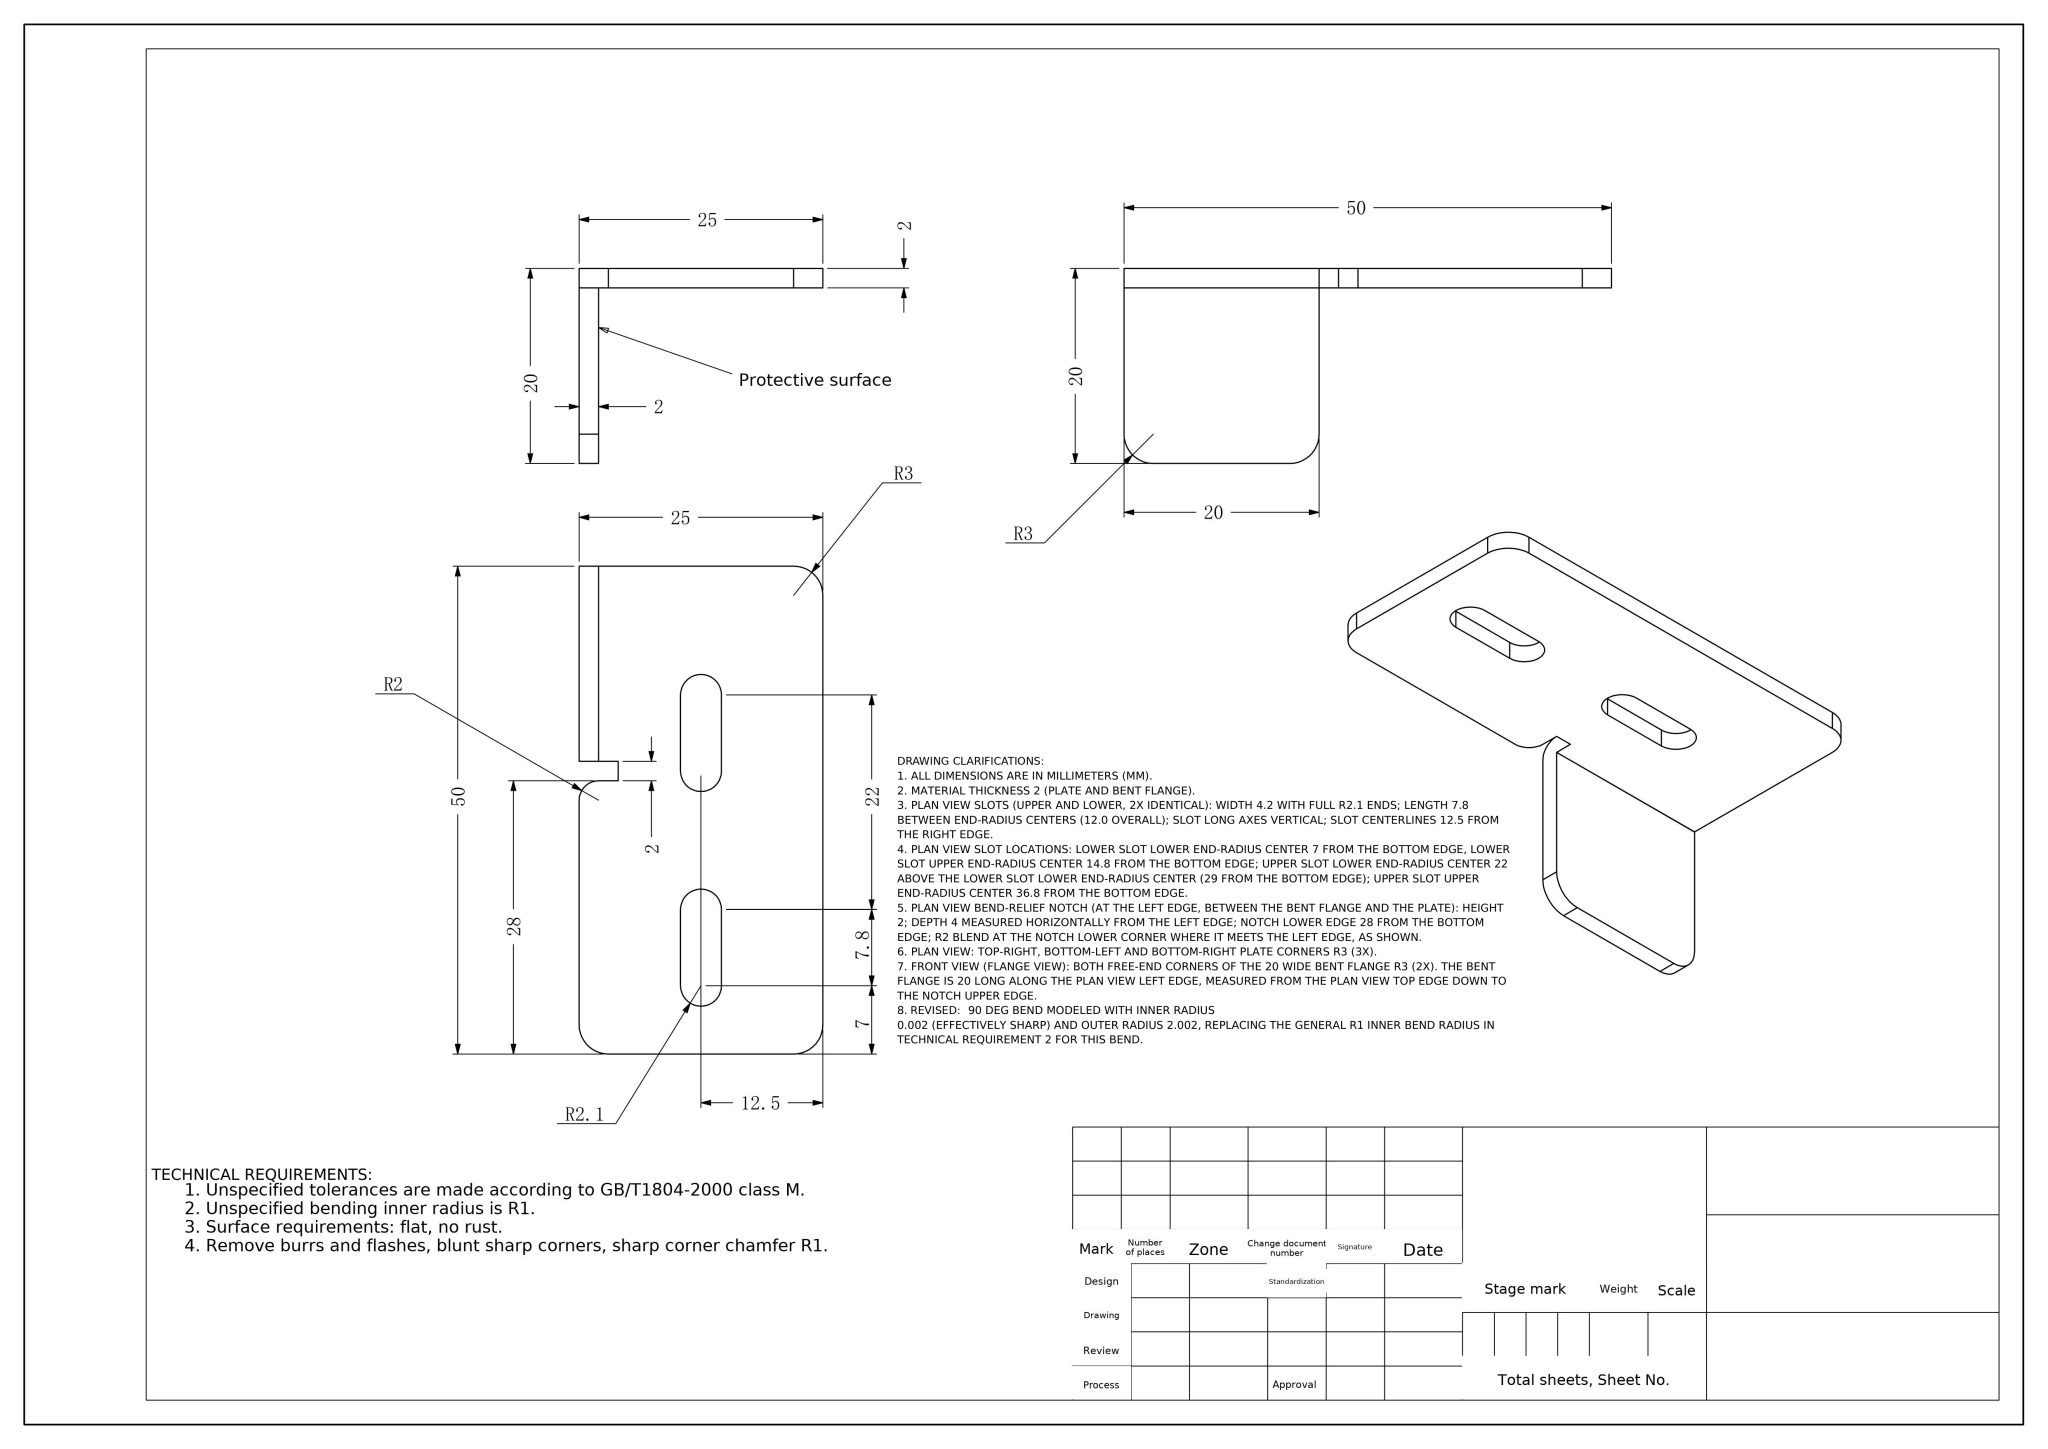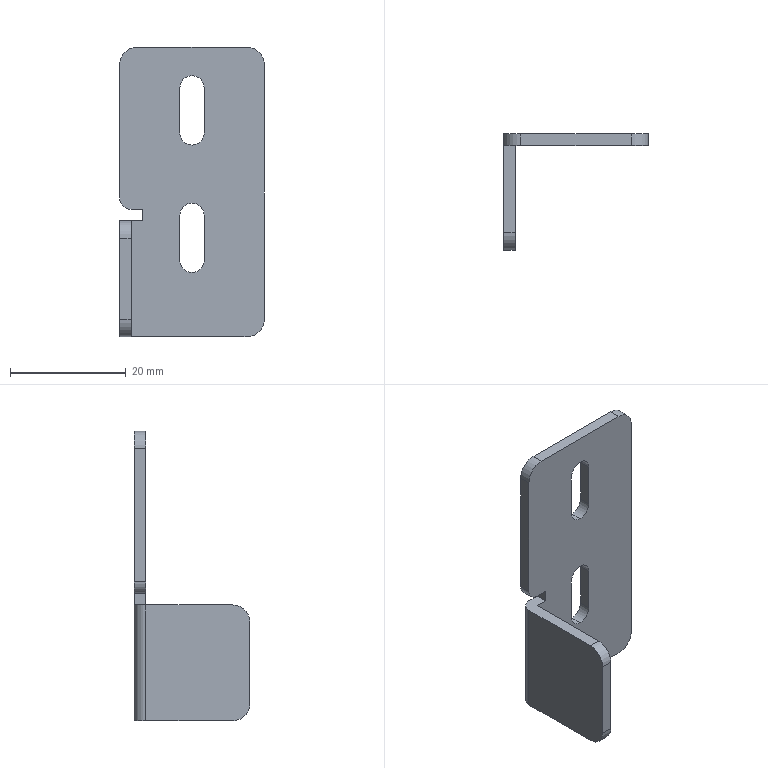Part | NX | mm | 1 solid | 30 faces | box 25 x 20 x 50 mm | volume 2979 mm3 | plane 16 | cylinder 14 | commonest cylinder face diameters 4.2 x6 6 x5 4.004 x1 0.004 x1 4 x1
STEP:
#1=COLOUR_RGB('',0.7529,0.7529,0.7529);
#2=FILL_AREA_STYLE_COLOUR('',#1);
#3=FILL_AREA_STYLE('',(#2));
#4=SURFACE_STYLE_FILL_AREA(#3);
#5=SURFACE_SIDE_STYLE('',(#4));
#6=SURFACE_STYLE_USAGE(.BOTH.,#5);
#7=PRESENTATION_STYLE_ASSIGNMENT((#6));
#8=CARTESIAN_POINT('',(16.5,16.3,46.764));
#9=VERTEX_POINT('',#8);
#10=CARTESIAN_POINT('',(18.6,16.3,48.864));
#11=VERTEX_POINT('',#10);
#12=CARTESIAN_POINT('',(16.5,16.3,48.864));
#13=DIRECTION('',(0.,-1.,0.));
#14=DIRECTION('',(0.,0.,-1.));
#15=AXIS2_PLACEMENT_3D('',#12,#13,#14);
#16=CIRCLE('',#15,2.1);
#17=EDGE_CURVE('',#9,#11,#16,.T.);
#18=ORIENTED_EDGE('',*,*,#17,.F.);
#19=CARTESIAN_POINT('',(16.5,14.3,46.764));
#20=VERTEX_POINT('',#19);
#21=CARTESIAN_POINT('',(16.5,16.3,46.764));
#22=DIRECTION('',(0.,-1.,0.));
#23=VECTOR('',#22,1000.);
#24=LINE('',#21,#23);
#25=EDGE_CURVE('',#9,#20,#24,.T.);
#26=ORIENTED_EDGE('',*,*,#25,.T.);
#27=CARTESIAN_POINT('',(18.6,14.3,48.864));
#28=VERTEX_POINT('',#27);
#29=CARTESIAN_POINT('',(16.5,14.3,48.864));
#30=DIRECTION('',(0.,-1.,0.));
#31=DIRECTION('',(0.,0.,-1.));
#32=AXIS2_PLACEMENT_3D('',#29,#30,#31);
#33=CIRCLE('',#32,2.1);
#34=EDGE_CURVE('',#20,#28,#33,.T.);
#35=ORIENTED_EDGE('',*,*,#34,.T.);
#36=CARTESIAN_POINT('',(18.6,16.3,48.864));
#37=DIRECTION('',(0.,1.,0.));
#38=VECTOR('',#37,1000.);
#39=LINE('',#36,#38);
#40=EDGE_CURVE('',#28,#11,#39,.T.);
#41=ORIENTED_EDGE('',*,*,#40,.T.);
#42=EDGE_LOOP('',(#18,#26,#35,#41));
#43=FACE_OUTER_BOUND('',#42,.T.);
#44=CARTESIAN_POINT('',(16.5,16.3,48.864));
#45=DIRECTION('',(0.,-1.,0.));
#46=DIRECTION('',(0.,0.,-1.));
#47=AXIS2_PLACEMENT_3D('',#44,#45,#46);
#48=CYLINDRICAL_SURFACE('',#47,2.1);
#49=ADVANCED_FACE('',(#43),#48,.F.);
#50=CARTESIAN_POINT('',(16.5,16.3,24.764));
#51=VERTEX_POINT('',#50);
#52=CARTESIAN_POINT('',(18.6,16.3,26.864));
#53=VERTEX_POINT('',#52);
#54=CARTESIAN_POINT('',(16.5,16.3,26.864));
#55=DIRECTION('',(0.,-1.,0.));
#56=DIRECTION('',(0.,0.,-1.));
#57=AXIS2_PLACEMENT_3D('',#54,#55,#56);
#58=CIRCLE('',#57,2.1);
#59=EDGE_CURVE('',#51,#53,#58,.T.);
#60=ORIENTED_EDGE('',*,*,#59,.F.);
#61=CARTESIAN_POINT('',(16.5,14.3,24.764));
#62=VERTEX_POINT('',#61);
#63=CARTESIAN_POINT('',(16.5,16.3,24.764));
#64=DIRECTION('',(0.,-1.,0.));
#65=VECTOR('',#64,1000.);
#66=LINE('',#63,#65);
#67=EDGE_CURVE('',#51,#62,#66,.T.);
#68=ORIENTED_EDGE('',*,*,#67,.T.);
#69=CARTESIAN_POINT('',(18.6,14.3,26.864));
#70=VERTEX_POINT('',#69);
#71=CARTESIAN_POINT('',(16.5,14.3,26.864));
#72=DIRECTION('',(0.,-1.,0.));
#73=DIRECTION('',(0.,0.,-1.));
#74=AXIS2_PLACEMENT_3D('',#71,#72,#73);
#75=CIRCLE('',#74,2.1);
#76=EDGE_CURVE('',#62,#70,#75,.T.);
#77=ORIENTED_EDGE('',*,*,#76,.T.);
#78=CARTESIAN_POINT('',(18.6,16.3,26.864));
#79=DIRECTION('',(0.,1.,0.));
#80=VECTOR('',#79,1000.);
#81=LINE('',#78,#80);
#82=EDGE_CURVE('',#70,#53,#81,.T.);
#83=ORIENTED_EDGE('',*,*,#82,.T.);
#84=EDGE_LOOP('',(#60,#68,#77,#83));
#85=FACE_OUTER_BOUND('',#84,.T.);
#86=CARTESIAN_POINT('',(16.5,16.3,26.864));
#87=DIRECTION('',(0.,-1.,0.));
#88=DIRECTION('',(0.,0.,-1.));
#89=AXIS2_PLACEMENT_3D('',#86,#87,#88);
#90=CYLINDRICAL_SURFACE('',#89,2.1);
#91=ADVANCED_FACE('',(#85),#90,.F.);
#92=CARTESIAN_POINT('',(4.,-0.7,33.664));
#93=VERTEX_POINT('',#92);
#94=CARTESIAN_POINT('',(4.,14.298,33.664));
#95=VERTEX_POINT('',#94);
#96=CARTESIAN_POINT('',(4.,14.818,33.664));
#97=DIRECTION('',(-0.,1.,-0.));
#98=VECTOR('',#97,1000.);
#99=LINE('',#96,#98);
#100=EDGE_CURVE('',#93,#95,#99,.T.);
#101=ORIENTED_EDGE('',*,*,#100,.F.);
#102=CARTESIAN_POINT('',(6.,-0.7,33.664));
#103=VERTEX_POINT('',#102);
#104=CARTESIAN_POINT('',(4.,-0.7,33.664));
#105=DIRECTION('',(1.,0.,0.));
#106=VECTOR('',#105,1000.);
#107=LINE('',#104,#106);
#108=EDGE_CURVE('',#93,#103,#107,.T.);
#109=ORIENTED_EDGE('',*,*,#108,.T.);
#110=CARTESIAN_POINT('',(6.,14.298,33.664));
#111=VERTEX_POINT('',#110);
#112=CARTESIAN_POINT('',(6.,14.818,33.664));
#113=DIRECTION('',(-0.,1.,-0.));
#114=VECTOR('',#113,1000.);
#115=LINE('',#112,#114);
#116=EDGE_CURVE('',#103,#111,#115,.T.);
#117=ORIENTED_EDGE('',*,*,#116,.T.);
#118=CARTESIAN_POINT('',(6.002,14.3,33.664));
#119=VERTEX_POINT('',#118);
#120=CARTESIAN_POINT('',(6.002,14.298,33.664));
#121=DIRECTION('',(0.,0.,1.));
#122=DIRECTION('',(1.,0.,0.));
#123=AXIS2_PLACEMENT_3D('',#120,#121,#122);
#124=CIRCLE('',#123,0.002);
#125=EDGE_CURVE('',#119,#111,#124,.T.);
#126=ORIENTED_EDGE('',*,*,#125,.F.);
#127=CARTESIAN_POINT('',(8.,14.3,33.664));
#128=VERTEX_POINT('',#127);
#129=CARTESIAN_POINT('',(4.,14.3,33.664));
#130=DIRECTION('',(-1.,0.,0.));
#131=VECTOR('',#130,1000.);
#132=LINE('',#129,#131);
#133=EDGE_CURVE('',#128,#119,#132,.T.);
#134=ORIENTED_EDGE('',*,*,#133,.F.);
#135=CARTESIAN_POINT('',(8.,16.3,33.664));
#136=VERTEX_POINT('',#135);
#137=CARTESIAN_POINT('',(8.,14.3,33.664));
#138=DIRECTION('',(0.,1.,0.));
#139=VECTOR('',#138,1000.);
#140=LINE('',#137,#139);
#141=EDGE_CURVE('',#128,#136,#140,.T.);
#142=ORIENTED_EDGE('',*,*,#141,.T.);
#143=CARTESIAN_POINT('',(6.002,16.3,33.664));
#144=VERTEX_POINT('',#143);
#145=CARTESIAN_POINT('',(4.,16.3,33.664));
#146=DIRECTION('',(-1.,0.,0.));
#147=VECTOR('',#146,1000.);
#148=LINE('',#145,#147);
#149=EDGE_CURVE('',#136,#144,#148,.T.);
#150=ORIENTED_EDGE('',*,*,#149,.T.);
#151=CARTESIAN_POINT('',(6.002,14.298,33.664));
#152=DIRECTION('',(0.,0.,1.));
#153=DIRECTION('',(0.,-1.,0.));
#154=AXIS2_PLACEMENT_3D('',#151,#152,#153);
#155=CIRCLE('',#154,2.002);
#156=EDGE_CURVE('',#144,#95,#155,.T.);
#157=ORIENTED_EDGE('',*,*,#156,.T.);
#158=EDGE_LOOP('',(#101,#109,#117,#126,#134,#142,#150,#157));
#159=FACE_OUTER_BOUND('',#158,.T.);
#160=CARTESIAN_POINT('',(4.,14.3,33.664));
#161=DIRECTION('',(0.,0.,-1.));
#162=DIRECTION('',(-1.,0.,0.));
#163=AXIS2_PLACEMENT_3D('',#160,#161,#162);
#164=PLANE('',#163);
#165=ADVANCED_FACE('',(#159),#164,.F.);
#166=CARTESIAN_POINT('',(6.002,16.3,13.664));
#167=VERTEX_POINT('',#166);
#168=CARTESIAN_POINT('',(26.,16.3,13.664));
#169=VERTEX_POINT('',#168);
#170=CARTESIAN_POINT('',(4.,16.3,13.664));
#171=DIRECTION('',(1.,0.,0.));
#172=VECTOR('',#171,1000.);
#173=LINE('',#170,#172);
#174=EDGE_CURVE('',#167,#169,#173,.T.);
#175=ORIENTED_EDGE('',*,*,#174,.T.);
#176=CARTESIAN_POINT('',(26.,14.3,13.664));
#177=VERTEX_POINT('',#176);
#178=CARTESIAN_POINT('',(26.,14.3,13.664));
#179=DIRECTION('',(0.,-1.,0.));
#180=VECTOR('',#179,1000.);
#181=LINE('',#178,#180);
#182=EDGE_CURVE('',#169,#177,#181,.T.);
#183=ORIENTED_EDGE('',*,*,#182,.T.);
#184=CARTESIAN_POINT('',(6.002,14.3,13.664));
#185=VERTEX_POINT('',#184);
#186=CARTESIAN_POINT('',(4.,14.3,13.664));
#187=DIRECTION('',(1.,0.,0.));
#188=VECTOR('',#187,1000.);
#189=LINE('',#186,#188);
#190=EDGE_CURVE('',#185,#177,#189,.T.);
#191=ORIENTED_EDGE('',*,*,#190,.F.);
#192=CARTESIAN_POINT('',(6.,14.298,13.664));
#193=VERTEX_POINT('',#192);
#194=CARTESIAN_POINT('',(6.002,14.298,13.664));
#195=DIRECTION('',(0.,0.,-1.));
#196=DIRECTION('',(1.,0.,0.));
#197=AXIS2_PLACEMENT_3D('',#194,#195,#196);
#198=CIRCLE('',#197,0.002);
#199=EDGE_CURVE('',#193,#185,#198,.T.);
#200=ORIENTED_EDGE('',*,*,#199,.F.);
#201=CARTESIAN_POINT('',(6.,-0.7,13.664));
#202=VERTEX_POINT('',#201);
#203=CARTESIAN_POINT('',(6.,14.818,13.664));
#204=DIRECTION('',(0.,-1.,0.));
#205=VECTOR('',#204,1000.);
#206=LINE('',#203,#205);
#207=EDGE_CURVE('',#193,#202,#206,.T.);
#208=ORIENTED_EDGE('',*,*,#207,.T.);
#209=CARTESIAN_POINT('',(4.,-0.7,13.664));
#210=VERTEX_POINT('',#209);
#211=CARTESIAN_POINT('',(4.,-0.7,13.664));
#212=DIRECTION('',(-1.,-0.,0.));
#213=VECTOR('',#212,1000.);
#214=LINE('',#211,#213);
#215=EDGE_CURVE('',#202,#210,#214,.T.);
#216=ORIENTED_EDGE('',*,*,#215,.T.);
#217=CARTESIAN_POINT('',(4.,14.298,13.664));
#218=VERTEX_POINT('',#217);
#219=CARTESIAN_POINT('',(4.,14.818,13.664));
#220=DIRECTION('',(0.,-1.,0.));
#221=VECTOR('',#220,1000.);
#222=LINE('',#219,#221);
#223=EDGE_CURVE('',#218,#210,#222,.T.);
#224=ORIENTED_EDGE('',*,*,#223,.F.);
#225=CARTESIAN_POINT('',(6.002,14.298,13.664));
#226=DIRECTION('',(0.,0.,-1.));
#227=DIRECTION('',(0.,-1.,0.));
#228=AXIS2_PLACEMENT_3D('',#225,#226,#227);
#229=CIRCLE('',#228,2.002);
#230=EDGE_CURVE('',#218,#167,#229,.T.);
#231=ORIENTED_EDGE('',*,*,#230,.T.);
#232=EDGE_LOOP('',(#175,#183,#191,#200,#208,#216,#224,#231));
#233=FACE_OUTER_BOUND('',#232,.T.);
#234=CARTESIAN_POINT('',(4.,14.3,13.664));
#235=DIRECTION('',(0.,0.,1.));
#236=DIRECTION('',(1.,0.,0.));
#237=AXIS2_PLACEMENT_3D('',#234,#235,#236);
#238=PLANE('',#237);
#239=ADVANCED_FACE('',(#233),#238,.F.);
#240=CARTESIAN_POINT('',(18.6,16.3,56.664));
#241=VERTEX_POINT('',#240);
#242=CARTESIAN_POINT('',(18.6,16.3,63.664));
#243=DIRECTION('',(0.,0.,1.));
#244=VECTOR('',#243,1000.);
#245=LINE('',#242,#244);
#246=EDGE_CURVE('',#11,#241,#245,.T.);
#247=ORIENTED_EDGE('',*,*,#246,.T.);
#248=CARTESIAN_POINT('',(14.4,16.3,56.664));
#249=VERTEX_POINT('',#248);
#250=CARTESIAN_POINT('',(16.5,16.3,56.664));
#251=DIRECTION('',(0.,-1.,0.));
#252=DIRECTION('',(0.,0.,-1.));
#253=AXIS2_PLACEMENT_3D('',#250,#251,#252);
#254=CIRCLE('',#253,2.1);
#255=EDGE_CURVE('',#241,#249,#254,.T.);
#256=ORIENTED_EDGE('',*,*,#255,.T.);
#257=CARTESIAN_POINT('',(14.4,16.3,48.864));
#258=VERTEX_POINT('',#257);
#259=CARTESIAN_POINT('',(14.4,16.3,63.664));
#260=DIRECTION('',(0.,0.,-1.));
#261=VECTOR('',#260,1000.);
#262=LINE('',#259,#261);
#263=EDGE_CURVE('',#249,#258,#262,.T.);
#264=ORIENTED_EDGE('',*,*,#263,.T.);
#265=CARTESIAN_POINT('',(16.5,16.3,48.864));
#266=DIRECTION('',(0.,-1.,0.));
#267=DIRECTION('',(0.,0.,-1.));
#268=AXIS2_PLACEMENT_3D('',#265,#266,#267);
#269=CIRCLE('',#268,2.1);
#270=EDGE_CURVE('',#258,#9,#269,.T.);
#271=ORIENTED_EDGE('',*,*,#270,.T.);
#272=ORIENTED_EDGE('',*,*,#17,.T.);
#273=EDGE_LOOP('',(#247,#256,#264,#271,#272));
#274=FACE_BOUND('',#273,.T.);
#275=CARTESIAN_POINT('',(18.6,16.3,34.664));
#276=VERTEX_POINT('',#275);
#277=CARTESIAN_POINT('',(18.6,16.3,63.664));
#278=DIRECTION('',(0.,0.,1.));
#279=VECTOR('',#278,1000.);
#280=LINE('',#277,#279);
#281=EDGE_CURVE('',#53,#276,#280,.T.);
#282=ORIENTED_EDGE('',*,*,#281,.T.);
#283=CARTESIAN_POINT('',(14.4,16.3,34.664));
#284=VERTEX_POINT('',#283);
#285=CARTESIAN_POINT('',(16.5,16.3,34.664));
#286=DIRECTION('',(0.,-1.,0.));
#287=DIRECTION('',(0.,0.,-1.));
#288=AXIS2_PLACEMENT_3D('',#285,#286,#287);
#289=CIRCLE('',#288,2.1);
#290=EDGE_CURVE('',#276,#284,#289,.T.);
#291=ORIENTED_EDGE('',*,*,#290,.T.);
#292=CARTESIAN_POINT('',(14.4,16.3,26.864));
#293=VERTEX_POINT('',#292);
#294=CARTESIAN_POINT('',(14.4,16.3,63.664));
#295=DIRECTION('',(0.,0.,-1.));
#296=VECTOR('',#295,1000.);
#297=LINE('',#294,#296);
#298=EDGE_CURVE('',#284,#293,#297,.T.);
#299=ORIENTED_EDGE('',*,*,#298,.T.);
#300=CARTESIAN_POINT('',(16.5,16.3,26.864));
#301=DIRECTION('',(0.,-1.,0.));
#302=DIRECTION('',(0.,0.,-1.));
#303=AXIS2_PLACEMENT_3D('',#300,#301,#302);
#304=CIRCLE('',#303,2.1);
#305=EDGE_CURVE('',#293,#51,#304,.T.);
#306=ORIENTED_EDGE('',*,*,#305,.T.);
#307=ORIENTED_EDGE('',*,*,#59,.T.);
#308=EDGE_LOOP('',(#282,#291,#299,#306,#307));
#309=FACE_BOUND('',#308,.T.);
#310=CARTESIAN_POINT('',(6.,16.3,35.664));
#311=VERTEX_POINT('',#310);
#312=CARTESIAN_POINT('',(8.,16.3,35.664));
#313=VERTEX_POINT('',#312);
#314=CARTESIAN_POINT('',(8.,16.3,35.664));
#315=DIRECTION('',(1.,0.,0.));
#316=VECTOR('',#315,1000.);
#317=LINE('',#314,#316);
#318=EDGE_CURVE('',#311,#313,#317,.T.);
#319=ORIENTED_EDGE('',*,*,#318,.F.);
#320=CARTESIAN_POINT('',(4.,16.3,37.664));
#321=VERTEX_POINT('',#320);
#322=CARTESIAN_POINT('',(6.,16.3,37.664));
#323=DIRECTION('',(0.,1.,0.));
#324=DIRECTION('',(0.,0.,-1.));
#325=AXIS2_PLACEMENT_3D('',#322,#323,#324);
#326=CIRCLE('',#325,2.);
#327=EDGE_CURVE('',#311,#321,#326,.T.);
#328=ORIENTED_EDGE('',*,*,#327,.T.);
#329=CARTESIAN_POINT('',(4.,16.3,60.664));
#330=VERTEX_POINT('',#329);
#331=CARTESIAN_POINT('',(4.,16.3,35.664));
#332=DIRECTION('',(0.,0.,-1.));
#333=VECTOR('',#332,1000.);
#334=LINE('',#331,#333);
#335=EDGE_CURVE('',#330,#321,#334,.T.);
#336=ORIENTED_EDGE('',*,*,#335,.F.);
#337=CARTESIAN_POINT('',(7.,16.3,63.664));
#338=VERTEX_POINT('',#337);
#339=CARTESIAN_POINT('',(7.,16.3,60.664));
#340=DIRECTION('',(0.,1.,0.));
#341=DIRECTION('',(0.,0.,-1.));
#342=AXIS2_PLACEMENT_3D('',#339,#340,#341);
#343=CIRCLE('',#342,3.);
#344=EDGE_CURVE('',#330,#338,#343,.T.);
#345=ORIENTED_EDGE('',*,*,#344,.T.);
#346=CARTESIAN_POINT('',(26.,16.3,63.664));
#347=VERTEX_POINT('',#346);
#348=CARTESIAN_POINT('',(4.,16.3,63.664));
#349=DIRECTION('',(-1.,0.,0.));
#350=VECTOR('',#349,1000.);
#351=LINE('',#348,#350);
#352=EDGE_CURVE('',#347,#338,#351,.T.);
#353=ORIENTED_EDGE('',*,*,#352,.F.);
#354=CARTESIAN_POINT('',(29.,16.3,60.664));
#355=VERTEX_POINT('',#354);
#356=CARTESIAN_POINT('',(26.,16.3,60.664));
#357=DIRECTION('',(0.,1.,0.));
#358=DIRECTION('',(0.,0.,-1.));
#359=AXIS2_PLACEMENT_3D('',#356,#357,#358);
#360=CIRCLE('',#359,3.);
#361=EDGE_CURVE('',#347,#355,#360,.T.);
#362=ORIENTED_EDGE('',*,*,#361,.T.);
#363=CARTESIAN_POINT('',(29.,16.3,16.664));
#364=VERTEX_POINT('',#363);
#365=CARTESIAN_POINT('',(29.,16.3,63.664));
#366=DIRECTION('',(-0.,0.,1.));
#367=VECTOR('',#366,1000.);
#368=LINE('',#365,#367);
#369=EDGE_CURVE('',#364,#355,#368,.T.);
#370=ORIENTED_EDGE('',*,*,#369,.F.);
#371=CARTESIAN_POINT('',(26.,16.3,16.664));
#372=DIRECTION('',(0.,1.,0.));
#373=DIRECTION('',(0.,0.,-1.));
#374=AXIS2_PLACEMENT_3D('',#371,#372,#373);
#375=CIRCLE('',#374,3.);
#376=EDGE_CURVE('',#364,#169,#375,.T.);
#377=ORIENTED_EDGE('',*,*,#376,.T.);
#378=ORIENTED_EDGE('',*,*,#174,.F.);
#379=CARTESIAN_POINT('',(6.002,16.3,13.664));
#380=DIRECTION('',(0.,0.,1.));
#381=VECTOR('',#380,1000.);
#382=LINE('',#379,#381);
#383=EDGE_CURVE('',#167,#144,#382,.T.);
#384=ORIENTED_EDGE('',*,*,#383,.T.);
#385=ORIENTED_EDGE('',*,*,#149,.F.);
#386=CARTESIAN_POINT('',(8.,16.3,33.664));
#387=DIRECTION('',(0.,0.,-1.));
#388=VECTOR('',#387,1000.);
#389=LINE('',#386,#388);
#390=EDGE_CURVE('',#313,#136,#389,.T.);
#391=ORIENTED_EDGE('',*,*,#390,.F.);
#392=EDGE_LOOP('',(#319,#328,#336,#345,#353,#362,#370,#377,#378,#384,#385,#391));
#393=FACE_OUTER_BOUND('',#392,.T.);
#394=CARTESIAN_POINT('',(29.,16.3,63.664));
#395=DIRECTION('',(0.,-1.,0.));
#396=DIRECTION('',(0.,0.,-1.));
#397=AXIS2_PLACEMENT_3D('',#394,#395,#396);
#398=PLANE('',#397);
#399=ADVANCED_FACE('',(#274,#309,#393),#398,.F.);
#400=CARTESIAN_POINT('',(29.,14.3,16.664));
#401=VERTEX_POINT('',#400);
#402=CARTESIAN_POINT('',(29.,14.3,60.664));
#403=VERTEX_POINT('',#402);
#404=CARTESIAN_POINT('',(29.,14.3,63.664));
#405=DIRECTION('',(-0.,0.,1.));
#406=VECTOR('',#405,1000.);
#407=LINE('',#404,#406);
#408=EDGE_CURVE('',#401,#403,#407,.T.);
#409=ORIENTED_EDGE('',*,*,#408,.F.);
#410=CARTESIAN_POINT('',(29.,14.3,16.664));
#411=DIRECTION('',(0.,1.,0.));
#412=VECTOR('',#411,1000.);
#413=LINE('',#410,#412);
#414=EDGE_CURVE('',#401,#364,#413,.T.);
#415=ORIENTED_EDGE('',*,*,#414,.T.);
#416=ORIENTED_EDGE('',*,*,#369,.T.);
#417=CARTESIAN_POINT('',(29.,14.3,60.664));
#418=DIRECTION('',(0.,-1.,0.));
#419=VECTOR('',#418,1000.);
#420=LINE('',#417,#419);
#421=EDGE_CURVE('',#355,#403,#420,.T.);
#422=ORIENTED_EDGE('',*,*,#421,.T.);
#423=EDGE_LOOP('',(#409,#415,#416,#422));
#424=FACE_OUTER_BOUND('',#423,.T.);
#425=CARTESIAN_POINT('',(29.,14.3,63.664));
#426=DIRECTION('',(-1.,0.,-0.));
#427=DIRECTION('',(-0.,0.,1.));
#428=AXIS2_PLACEMENT_3D('',#425,#426,#427);
#429=PLANE('',#428);
#430=ADVANCED_FACE('',(#424),#429,.F.);
#431=CARTESIAN_POINT('',(26.,14.3,63.664));
#432=VERTEX_POINT('',#431);
#433=CARTESIAN_POINT('',(7.,14.3,63.664));
#434=VERTEX_POINT('',#433);
#435=CARTESIAN_POINT('',(4.,14.3,63.664));
#436=DIRECTION('',(-1.,0.,0.));
#437=VECTOR('',#436,1000.);
#438=LINE('',#435,#437);
#439=EDGE_CURVE('',#432,#434,#438,.T.);
#440=ORIENTED_EDGE('',*,*,#439,.F.);
#441=CARTESIAN_POINT('',(26.,14.3,63.664));
#442=DIRECTION('',(0.,1.,0.));
#443=VECTOR('',#442,1000.);
#444=LINE('',#441,#443);
#445=EDGE_CURVE('',#432,#347,#444,.T.);
#446=ORIENTED_EDGE('',*,*,#445,.T.);
#447=ORIENTED_EDGE('',*,*,#352,.T.);
#448=CARTESIAN_POINT('',(7.,14.3,63.664));
#449=DIRECTION('',(0.,-1.,0.));
#450=VECTOR('',#449,1000.);
#451=LINE('',#448,#450);
#452=EDGE_CURVE('',#338,#434,#451,.T.);
#453=ORIENTED_EDGE('',*,*,#452,.T.);
#454=EDGE_LOOP('',(#440,#446,#447,#453));
#455=FACE_OUTER_BOUND('',#454,.T.);
#456=CARTESIAN_POINT('',(4.,14.3,63.664));
#457=DIRECTION('',(0.,0.,-1.));
#458=DIRECTION('',(-1.,0.,0.));
#459=AXIS2_PLACEMENT_3D('',#456,#457,#458);
#460=PLANE('',#459);
#461=ADVANCED_FACE('',(#455),#460,.F.);
#462=ORIENTED_EDGE('',*,*,#335,.T.);
#463=CARTESIAN_POINT('',(4.,14.3,37.664));
#464=VERTEX_POINT('',#463);
#465=CARTESIAN_POINT('',(4.,14.3,37.664));
#466=DIRECTION('',(0.,-1.,0.));
#467=VECTOR('',#466,1000.);
#468=LINE('',#465,#467);
#469=EDGE_CURVE('',#321,#464,#468,.T.);
#470=ORIENTED_EDGE('',*,*,#469,.T.);
#471=CARTESIAN_POINT('',(4.,14.3,60.664));
#472=VERTEX_POINT('',#471);
#473=CARTESIAN_POINT('',(4.,14.3,35.664));
#474=DIRECTION('',(0.,0.,-1.));
#475=VECTOR('',#474,1000.);
#476=LINE('',#473,#475);
#477=EDGE_CURVE('',#472,#464,#476,.T.);
#478=ORIENTED_EDGE('',*,*,#477,.F.);
#479=CARTESIAN_POINT('',(4.,14.3,60.664));
#480=DIRECTION('',(0.,1.,0.));
#481=VECTOR('',#480,1000.);
#482=LINE('',#479,#481);
#483=EDGE_CURVE('',#472,#330,#482,.T.);
#484=ORIENTED_EDGE('',*,*,#483,.T.);
#485=EDGE_LOOP('',(#462,#470,#478,#484));
#486=FACE_OUTER_BOUND('',#485,.T.);
#487=CARTESIAN_POINT('',(4.,14.3,35.664));
#488=DIRECTION('',(1.,0.,0.));
#489=DIRECTION('',(0.,0.,-1.));
#490=AXIS2_PLACEMENT_3D('',#487,#488,#489);
#491=PLANE('',#490);
#492=ADVANCED_FACE('',(#486),#491,.F.);
#493=CARTESIAN_POINT('',(6.,14.3,35.664));
#494=VERTEX_POINT('',#493);
#495=CARTESIAN_POINT('',(8.,14.3,35.664));
#496=VERTEX_POINT('',#495);
#497=CARTESIAN_POINT('',(8.,14.3,35.664));
#498=DIRECTION('',(1.,0.,0.));
#499=VECTOR('',#498,1000.);
#500=LINE('',#497,#499);
#501=EDGE_CURVE('',#494,#496,#500,.T.);
#502=ORIENTED_EDGE('',*,*,#501,.F.);
#503=CARTESIAN_POINT('',(6.,14.3,35.664));
#504=DIRECTION('',(0.,1.,0.));
#505=VECTOR('',#504,1000.);
#506=LINE('',#503,#505);
#507=EDGE_CURVE('',#494,#311,#506,.T.);
#508=ORIENTED_EDGE('',*,*,#507,.T.);
#509=ORIENTED_EDGE('',*,*,#318,.T.);
#510=CARTESIAN_POINT('',(8.,14.3,35.664));
#511=DIRECTION('',(0.,1.,0.));
#512=VECTOR('',#511,1000.);
#513=LINE('',#510,#512);
#514=EDGE_CURVE('',#496,#313,#513,.T.);
#515=ORIENTED_EDGE('',*,*,#514,.F.);
#516=EDGE_LOOP('',(#502,#508,#509,#515));
#517=FACE_OUTER_BOUND('',#516,.T.);
#518=CARTESIAN_POINT('',(8.,14.3,35.664));
#519=DIRECTION('',(0.,0.,1.));
#520=DIRECTION('',(1.,0.,0.));
#521=AXIS2_PLACEMENT_3D('',#518,#519,#520);
#522=PLANE('',#521);
#523=ADVANCED_FACE('',(#517),#522,.F.);
#524=ORIENTED_EDGE('',*,*,#390,.T.);
#525=ORIENTED_EDGE('',*,*,#141,.F.);
#526=CARTESIAN_POINT('',(8.,14.3,33.664));
#527=DIRECTION('',(0.,0.,-1.));
#528=VECTOR('',#527,1000.);
#529=LINE('',#526,#528);
#530=EDGE_CURVE('',#496,#128,#529,.T.);
#531=ORIENTED_EDGE('',*,*,#530,.F.);
#532=ORIENTED_EDGE('',*,*,#514,.T.);
#533=EDGE_LOOP('',(#524,#525,#531,#532));
#534=FACE_OUTER_BOUND('',#533,.T.);
#535=CARTESIAN_POINT('',(8.,14.3,33.664));
#536=DIRECTION('',(1.,0.,0.));
#537=DIRECTION('',(0.,0.,-1.));
#538=AXIS2_PLACEMENT_3D('',#535,#536,#537);
#539=PLANE('',#538);
#540=ADVANCED_FACE('',(#534),#539,.F.);
#541=CARTESIAN_POINT('',(18.6,14.3,56.664));
#542=VERTEX_POINT('',#541);
#543=CARTESIAN_POINT('',(14.4,14.3,56.664));
#544=VERTEX_POINT('',#543);
#545=CARTESIAN_POINT('',(16.5,14.3,56.664));
#546=DIRECTION('',(0.,-1.,0.));
#547=DIRECTION('',(0.,0.,-1.));
#548=AXIS2_PLACEMENT_3D('',#545,#546,#547);
#549=CIRCLE('',#548,2.1);
#550=EDGE_CURVE('',#542,#544,#549,.T.);
#551=ORIENTED_EDGE('',*,*,#550,.F.);
#552=CARTESIAN_POINT('',(18.6,14.3,63.664));
#553=DIRECTION('',(0.,0.,1.));
#554=VECTOR('',#553,1000.);
#555=LINE('',#552,#554);
#556=EDGE_CURVE('',#28,#542,#555,.T.);
#557=ORIENTED_EDGE('',*,*,#556,.F.);
#558=ORIENTED_EDGE('',*,*,#34,.F.);
#559=CARTESIAN_POINT('',(14.4,14.3,48.864));
#560=VERTEX_POINT('',#559);
#561=CARTESIAN_POINT('',(16.5,14.3,48.864));
#562=DIRECTION('',(0.,-1.,0.));
#563=DIRECTION('',(0.,0.,-1.));
#564=AXIS2_PLACEMENT_3D('',#561,#562,#563);
#565=CIRCLE('',#564,2.1);
#566=EDGE_CURVE('',#560,#20,#565,.T.);
#567=ORIENTED_EDGE('',*,*,#566,.F.);
#568=CARTESIAN_POINT('',(14.4,14.3,63.664));
#569=DIRECTION('',(0.,0.,-1.));
#570=VECTOR('',#569,1000.);
#571=LINE('',#568,#570);
#572=EDGE_CURVE('',#544,#560,#571,.T.);
#573=ORIENTED_EDGE('',*,*,#572,.F.);
#574=EDGE_LOOP('',(#551,#557,#558,#567,#573));
#575=FACE_BOUND('',#574,.T.);
#576=CARTESIAN_POINT('',(18.6,14.3,34.664));
#577=VERTEX_POINT('',#576);
#578=CARTESIAN_POINT('',(14.4,14.3,34.664));
#579=VERTEX_POINT('',#578);
#580=CARTESIAN_POINT('',(16.5,14.3,34.664));
#581=DIRECTION('',(0.,-1.,0.));
#582=DIRECTION('',(0.,0.,-1.));
#583=AXIS2_PLACEMENT_3D('',#580,#581,#582);
#584=CIRCLE('',#583,2.1);
#585=EDGE_CURVE('',#577,#579,#584,.T.);
#586=ORIENTED_EDGE('',*,*,#585,.F.);
#587=CARTESIAN_POINT('',(18.6,14.3,63.664));
#588=DIRECTION('',(0.,0.,1.));
#589=VECTOR('',#588,1000.);
#590=LINE('',#587,#589);
#591=EDGE_CURVE('',#70,#577,#590,.T.);
#592=ORIENTED_EDGE('',*,*,#591,.F.);
#593=ORIENTED_EDGE('',*,*,#76,.F.);
#594=CARTESIAN_POINT('',(14.4,14.3,26.864));
#595=VERTEX_POINT('',#594);
#596=CARTESIAN_POINT('',(16.5,14.3,26.864));
#597=DIRECTION('',(0.,-1.,0.));
#598=DIRECTION('',(0.,0.,-1.));
#599=AXIS2_PLACEMENT_3D('',#596,#597,#598);
#600=CIRCLE('',#599,2.1);
#601=EDGE_CURVE('',#595,#62,#600,.T.);
#602=ORIENTED_EDGE('',*,*,#601,.F.);
#603=CARTESIAN_POINT('',(14.4,14.3,63.664));
#604=DIRECTION('',(0.,0.,-1.));
#605=VECTOR('',#604,1000.);
#606=LINE('',#603,#605);
#607=EDGE_CURVE('',#579,#595,#606,.T.);
#608=ORIENTED_EDGE('',*,*,#607,.F.);
#609=EDGE_LOOP('',(#586,#592,#593,#602,#608));
#610=FACE_BOUND('',#609,.T.);
#611=ORIENTED_EDGE('',*,*,#477,.T.);
#612=CARTESIAN_POINT('',(6.,14.3,37.664));
#613=DIRECTION('',(0.,-1.,0.));
#614=DIRECTION('',(0.,0.,-1.));
#615=AXIS2_PLACEMENT_3D('',#612,#613,#614);
#616=CIRCLE('',#615,2.);
#617=EDGE_CURVE('',#464,#494,#616,.T.);
#618=ORIENTED_EDGE('',*,*,#617,.T.);
#619=ORIENTED_EDGE('',*,*,#501,.T.);
#620=ORIENTED_EDGE('',*,*,#530,.T.);
#621=ORIENTED_EDGE('',*,*,#133,.T.);
#622=CARTESIAN_POINT('',(6.002,14.3,13.664));
#623=DIRECTION('',(0.,0.,1.));
#624=VECTOR('',#623,1000.);
#625=LINE('',#622,#624);
#626=EDGE_CURVE('',#185,#119,#625,.T.);
#627=ORIENTED_EDGE('',*,*,#626,.F.);
#628=ORIENTED_EDGE('',*,*,#190,.T.);
#629=CARTESIAN_POINT('',(26.,14.3,16.664));
#630=DIRECTION('',(0.,-1.,0.));
#631=DIRECTION('',(0.,0.,-1.));
#632=AXIS2_PLACEMENT_3D('',#629,#630,#631);
#633=CIRCLE('',#632,3.);
#634=EDGE_CURVE('',#177,#401,#633,.T.);
#635=ORIENTED_EDGE('',*,*,#634,.T.);
#636=ORIENTED_EDGE('',*,*,#408,.T.);
#637=CARTESIAN_POINT('',(26.,14.3,60.664));
#638=DIRECTION('',(0.,-1.,0.));
#639=DIRECTION('',(0.,0.,-1.));
#640=AXIS2_PLACEMENT_3D('',#637,#638,#639);
#641=CIRCLE('',#640,3.);
#642=EDGE_CURVE('',#403,#432,#641,.T.);
#643=ORIENTED_EDGE('',*,*,#642,.T.);
#644=ORIENTED_EDGE('',*,*,#439,.T.);
#645=CARTESIAN_POINT('',(7.,14.3,60.664));
#646=DIRECTION('',(0.,-1.,0.));
#647=DIRECTION('',(0.,0.,-1.));
#648=AXIS2_PLACEMENT_3D('',#645,#646,#647);
#649=CIRCLE('',#648,3.);
#650=EDGE_CURVE('',#434,#472,#649,.T.);
#651=ORIENTED_EDGE('',*,*,#650,.T.);
#652=EDGE_LOOP('',(#611,#618,#619,#620,#621,#627,#628,#635,#636,#643,#644,#651));
#653=FACE_OUTER_BOUND('',#652,.T.);
#654=CARTESIAN_POINT('',(29.,14.3,63.664));
#655=DIRECTION('',(0.,-1.,0.));
#656=DIRECTION('',(0.,0.,-1.));
#657=AXIS2_PLACEMENT_3D('',#654,#655,#656);
#658=PLANE('',#657);
#659=ADVANCED_FACE('',(#575,#610,#653),#658,.T.);
#660=CARTESIAN_POINT('',(4.,-3.7,16.664));
#661=VERTEX_POINT('',#660);
#662=CARTESIAN_POINT('',(4.,-3.7,30.664));
#663=VERTEX_POINT('',#662);
#664=CARTESIAN_POINT('',(4.,-3.7,13.664));
#665=DIRECTION('',(0.,0.,1.));
#666=VECTOR('',#665,1000.);
#667=LINE('',#664,#666);
#668=EDGE_CURVE('',#661,#663,#667,.T.);
#669=ORIENTED_EDGE('',*,*,#668,.T.);
#670=CARTESIAN_POINT('',(4.,-0.7,30.664));
#671=DIRECTION('',(-1.,-0.,0.));
#672=DIRECTION('',(0.,-1.,0.));
#673=AXIS2_PLACEMENT_3D('',#670,#671,#672);
#674=CIRCLE('',#673,3.);
#675=EDGE_CURVE('',#663,#93,#674,.T.);
#676=ORIENTED_EDGE('',*,*,#675,.T.);
#677=ORIENTED_EDGE('',*,*,#100,.T.);
#678=CARTESIAN_POINT('',(4.,14.298,33.664));
#679=DIRECTION('',(0.,0.,-1.));
#680=VECTOR('',#679,1000.);
#681=LINE('',#678,#680);
#682=EDGE_CURVE('',#95,#218,#681,.T.);
#683=ORIENTED_EDGE('',*,*,#682,.T.);
#684=ORIENTED_EDGE('',*,*,#223,.T.);
#685=CARTESIAN_POINT('',(4.,-0.7,16.664));
#686=DIRECTION('',(-1.,-0.,0.));
#687=DIRECTION('',(0.,-1.,0.));
#688=AXIS2_PLACEMENT_3D('',#685,#686,#687);
#689=CIRCLE('',#688,3.);
#690=EDGE_CURVE('',#210,#661,#689,.T.);
#691=ORIENTED_EDGE('',*,*,#690,.T.);
#692=EDGE_LOOP('',(#669,#676,#677,#683,#684,#691));
#693=FACE_OUTER_BOUND('',#692,.T.);
#694=CARTESIAN_POINT('',(4.,14.818,33.664));
#695=DIRECTION('',(-1.,-0.,0.));
#696=DIRECTION('',(0.,-1.,0.));
#697=AXIS2_PLACEMENT_3D('',#694,#695,#696);
#698=PLANE('',#697);
#699=ADVANCED_FACE('',(#693),#698,.T.);
#700=ORIENTED_EDGE('',*,*,#116,.F.);
#701=CARTESIAN_POINT('',(6.,-3.7,30.664));
#702=VERTEX_POINT('',#701);
#703=CARTESIAN_POINT('',(6.,-0.7,30.664));
#704=DIRECTION('',(1.,0.,0.));
#705=DIRECTION('',(0.,-1.,0.));
#706=AXIS2_PLACEMENT_3D('',#703,#704,#705);
#707=CIRCLE('',#706,3.);
#708=EDGE_CURVE('',#103,#702,#707,.T.);
#709=ORIENTED_EDGE('',*,*,#708,.T.);
#710=CARTESIAN_POINT('',(6.,-3.7,16.664));
#711=VERTEX_POINT('',#710);
#712=CARTESIAN_POINT('',(6.,-3.7,13.664));
#713=DIRECTION('',(0.,0.,1.));
#714=VECTOR('',#713,1000.);
#715=LINE('',#712,#714);
#716=EDGE_CURVE('',#711,#702,#715,.T.);
#717=ORIENTED_EDGE('',*,*,#716,.F.);
#718=CARTESIAN_POINT('',(6.,-0.7,16.664));
#719=DIRECTION('',(1.,0.,0.));
#720=DIRECTION('',(0.,-1.,0.));
#721=AXIS2_PLACEMENT_3D('',#718,#719,#720);
#722=CIRCLE('',#721,3.);
#723=EDGE_CURVE('',#711,#202,#722,.T.);
#724=ORIENTED_EDGE('',*,*,#723,.T.);
#725=ORIENTED_EDGE('',*,*,#207,.F.);
#726=CARTESIAN_POINT('',(6.,14.298,33.664));
#727=DIRECTION('',(0.,0.,-1.));
#728=VECTOR('',#727,1000.);
#729=LINE('',#726,#728);
#730=EDGE_CURVE('',#111,#193,#729,.T.);
#731=ORIENTED_EDGE('',*,*,#730,.F.);
#732=EDGE_LOOP('',(#700,#709,#717,#724,#725,#731));
#733=FACE_OUTER_BOUND('',#732,.T.);
#734=CARTESIAN_POINT('',(6.,14.818,33.664));
#735=DIRECTION('',(-1.,-0.,0.));
#736=DIRECTION('',(0.,-1.,0.));
#737=AXIS2_PLACEMENT_3D('',#734,#735,#736);
#738=PLANE('',#737);
#739=ADVANCED_FACE('',(#733),#738,.F.);
#740=ORIENTED_EDGE('',*,*,#716,.T.);
#741=CARTESIAN_POINT('',(4.,-3.7,30.664));
#742=DIRECTION('',(-1.,-0.,0.));
#743=VECTOR('',#742,1000.);
#744=LINE('',#741,#743);
#745=EDGE_CURVE('',#702,#663,#744,.T.);
#746=ORIENTED_EDGE('',*,*,#745,.T.);
#747=ORIENTED_EDGE('',*,*,#668,.F.);
#748=CARTESIAN_POINT('',(4.,-3.7,16.664));
#749=DIRECTION('',(1.,0.,0.));
#750=VECTOR('',#749,1000.);
#751=LINE('',#748,#750);
#752=EDGE_CURVE('',#661,#711,#751,.T.);
#753=ORIENTED_EDGE('',*,*,#752,.T.);
#754=EDGE_LOOP('',(#740,#746,#747,#753));
#755=FACE_OUTER_BOUND('',#754,.T.);
#756=CARTESIAN_POINT('',(4.,-3.7,13.664));
#757=DIRECTION('',(-0.,1.,0.));
#758=DIRECTION('',(-1.,-0.,0.));
#759=AXIS2_PLACEMENT_3D('',#756,#757,#758);
#760=PLANE('',#759);
#761=ADVANCED_FACE('',(#755),#760,.F.);
#762=ORIENTED_EDGE('',*,*,#383,.F.);
#763=ORIENTED_EDGE('',*,*,#230,.F.);
#764=ORIENTED_EDGE('',*,*,#682,.F.);
#765=ORIENTED_EDGE('',*,*,#156,.F.);
#766=EDGE_LOOP('',(#762,#763,#764,#765));
#767=FACE_OUTER_BOUND('',#766,.T.);
#768=CARTESIAN_POINT('',(6.002,14.298,13.664));
#769=DIRECTION('',(0.,0.,1.));
#770=DIRECTION('',(0.,-1.,0.));
#771=AXIS2_PLACEMENT_3D('',#768,#769,#770);
#772=CYLINDRICAL_SURFACE('',#771,2.002);
#773=ADVANCED_FACE('',(#767),#772,.T.);
#774=ORIENTED_EDGE('',*,*,#626,.T.);
#775=ORIENTED_EDGE('',*,*,#125,.T.);
#776=ORIENTED_EDGE('',*,*,#730,.T.);
#777=ORIENTED_EDGE('',*,*,#199,.T.);
#778=EDGE_LOOP('',(#774,#775,#776,#777));
#779=FACE_OUTER_BOUND('',#778,.T.);
#780=CARTESIAN_POINT('',(6.002,14.298,13.664));
#781=DIRECTION('',(0.,0.,1.));
#782=DIRECTION('',(0.,-1.,0.));
#783=AXIS2_PLACEMENT_3D('',#780,#781,#782);
#784=CYLINDRICAL_SURFACE('',#783,0.002);
#785=ADVANCED_FACE('',(#779),#784,.F.);
#786=CARTESIAN_POINT('',(14.4,16.3,34.664));
#787=DIRECTION('',(0.,1.,0.));
#788=VECTOR('',#787,1000.);
#789=LINE('',#786,#788);
#790=EDGE_CURVE('',#579,#284,#789,.T.);
#791=ORIENTED_EDGE('',*,*,#790,.T.);
#792=ORIENTED_EDGE('',*,*,#290,.F.);
#793=CARTESIAN_POINT('',(18.6,16.3,34.664));
#794=DIRECTION('',(0.,1.,0.));
#795=VECTOR('',#794,1000.);
#796=LINE('',#793,#795);
#797=EDGE_CURVE('',#577,#276,#796,.T.);
#798=ORIENTED_EDGE('',*,*,#797,.F.);
#799=ORIENTED_EDGE('',*,*,#585,.T.);
#800=EDGE_LOOP('',(#791,#792,#798,#799));
#801=FACE_OUTER_BOUND('',#800,.T.);
#802=CARTESIAN_POINT('',(16.5,16.3,34.664));
#803=DIRECTION('',(0.,-1.,0.));
#804=DIRECTION('',(0.,0.,-1.));
#805=AXIS2_PLACEMENT_3D('',#802,#803,#804);
#806=CYLINDRICAL_SURFACE('',#805,2.1);
#807=ADVANCED_FACE('',(#801),#806,.F.);
#808=ORIENTED_EDGE('',*,*,#797,.T.);
#809=ORIENTED_EDGE('',*,*,#281,.F.);
#810=ORIENTED_EDGE('',*,*,#82,.F.);
#811=ORIENTED_EDGE('',*,*,#591,.T.);
#812=EDGE_LOOP('',(#808,#809,#810,#811));
#813=FACE_OUTER_BOUND('',#812,.T.);
#814=CARTESIAN_POINT('',(18.6,16.3,63.664));
#815=DIRECTION('',(1.,0.,0.));
#816=DIRECTION('',(0.,0.,1.));
#817=AXIS2_PLACEMENT_3D('',#814,#815,#816);
#818=PLANE('',#817);
#819=ADVANCED_FACE('',(#813),#818,.F.);
#820=ORIENTED_EDGE('',*,*,#67,.F.);
#821=ORIENTED_EDGE('',*,*,#305,.F.);
#822=CARTESIAN_POINT('',(14.4,16.3,26.864));
#823=DIRECTION('',(0.,1.,0.));
#824=VECTOR('',#823,1000.);
#825=LINE('',#822,#824);
#826=EDGE_CURVE('',#595,#293,#825,.T.);
#827=ORIENTED_EDGE('',*,*,#826,.F.);
#828=ORIENTED_EDGE('',*,*,#601,.T.);
#829=EDGE_LOOP('',(#820,#821,#827,#828));
#830=FACE_OUTER_BOUND('',#829,.T.);
#831=CARTESIAN_POINT('',(16.5,16.3,26.864));
#832=DIRECTION('',(0.,-1.,0.));
#833=DIRECTION('',(0.,0.,-1.));
#834=AXIS2_PLACEMENT_3D('',#831,#832,#833);
#835=CYLINDRICAL_SURFACE('',#834,2.1);
#836=ADVANCED_FACE('',(#830),#835,.F.);
#837=ORIENTED_EDGE('',*,*,#607,.T.);
#838=ORIENTED_EDGE('',*,*,#826,.T.);
#839=ORIENTED_EDGE('',*,*,#298,.F.);
#840=ORIENTED_EDGE('',*,*,#790,.F.);
#841=EDGE_LOOP('',(#837,#838,#839,#840));
#842=FACE_OUTER_BOUND('',#841,.T.);
#843=CARTESIAN_POINT('',(14.4,16.3,63.664));
#844=DIRECTION('',(-1.,0.,0.));
#845=DIRECTION('',(0.,0.,-1.));
#846=AXIS2_PLACEMENT_3D('',#843,#844,#845);
#847=PLANE('',#846);
#848=ADVANCED_FACE('',(#842),#847,.F.);
#849=CARTESIAN_POINT('',(14.4,16.3,56.664));
#850=DIRECTION('',(0.,1.,0.));
#851=VECTOR('',#850,1000.);
#852=LINE('',#849,#851);
#853=EDGE_CURVE('',#544,#249,#852,.T.);
#854=ORIENTED_EDGE('',*,*,#853,.T.);
#855=ORIENTED_EDGE('',*,*,#255,.F.);
#856=CARTESIAN_POINT('',(18.6,16.3,56.664));
#857=DIRECTION('',(0.,1.,0.));
#858=VECTOR('',#857,1000.);
#859=LINE('',#856,#858);
#860=EDGE_CURVE('',#542,#241,#859,.T.);
#861=ORIENTED_EDGE('',*,*,#860,.F.);
#862=ORIENTED_EDGE('',*,*,#550,.T.);
#863=EDGE_LOOP('',(#854,#855,#861,#862));
#864=FACE_OUTER_BOUND('',#863,.T.);
#865=CARTESIAN_POINT('',(16.5,16.3,56.664));
#866=DIRECTION('',(0.,-1.,0.));
#867=DIRECTION('',(0.,0.,-1.));
#868=AXIS2_PLACEMENT_3D('',#865,#866,#867);
#869=CYLINDRICAL_SURFACE('',#868,2.1);
#870=ADVANCED_FACE('',(#864),#869,.F.);
#871=ORIENTED_EDGE('',*,*,#860,.T.);
#872=ORIENTED_EDGE('',*,*,#246,.F.);
#873=ORIENTED_EDGE('',*,*,#40,.F.);
#874=ORIENTED_EDGE('',*,*,#556,.T.);
#875=EDGE_LOOP('',(#871,#872,#873,#874));
#876=FACE_OUTER_BOUND('',#875,.T.);
#877=CARTESIAN_POINT('',(18.6,16.3,63.664));
#878=DIRECTION('',(1.,0.,0.));
#879=DIRECTION('',(0.,0.,1.));
#880=AXIS2_PLACEMENT_3D('',#877,#878,#879);
#881=PLANE('',#880);
#882=ADVANCED_FACE('',(#876),#881,.F.);
#883=ORIENTED_EDGE('',*,*,#25,.F.);
#884=ORIENTED_EDGE('',*,*,#270,.F.);
#885=CARTESIAN_POINT('',(14.4,16.3,48.864));
#886=DIRECTION('',(0.,1.,0.));
#887=VECTOR('',#886,1000.);
#888=LINE('',#885,#887);
#889=EDGE_CURVE('',#560,#258,#888,.T.);
#890=ORIENTED_EDGE('',*,*,#889,.F.);
#891=ORIENTED_EDGE('',*,*,#566,.T.);
#892=EDGE_LOOP('',(#883,#884,#890,#891));
#893=FACE_OUTER_BOUND('',#892,.T.);
#894=CARTESIAN_POINT('',(16.5,16.3,48.864));
#895=DIRECTION('',(0.,-1.,0.));
#896=DIRECTION('',(0.,0.,-1.));
#897=AXIS2_PLACEMENT_3D('',#894,#895,#896);
#898=CYLINDRICAL_SURFACE('',#897,2.1);
#899=ADVANCED_FACE('',(#893),#898,.F.);
#900=ORIENTED_EDGE('',*,*,#572,.T.);
#901=ORIENTED_EDGE('',*,*,#889,.T.);
#902=ORIENTED_EDGE('',*,*,#263,.F.);
#903=ORIENTED_EDGE('',*,*,#853,.F.);
#904=EDGE_LOOP('',(#900,#901,#902,#903));
#905=FACE_OUTER_BOUND('',#904,.T.);
#906=CARTESIAN_POINT('',(14.4,16.3,63.664));
#907=DIRECTION('',(-1.,0.,0.));
#908=DIRECTION('',(0.,0.,-1.));
#909=AXIS2_PLACEMENT_3D('',#906,#907,#908);
#910=PLANE('',#909);
#911=ADVANCED_FACE('',(#905),#910,.F.);
#912=ORIENTED_EDGE('',*,*,#675,.F.);
#913=ORIENTED_EDGE('',*,*,#745,.F.);
#914=ORIENTED_EDGE('',*,*,#708,.F.);
#915=ORIENTED_EDGE('',*,*,#108,.F.);
#916=EDGE_LOOP('',(#912,#913,#914,#915));
#917=FACE_OUTER_BOUND('',#916,.T.);
#918=CARTESIAN_POINT('',(4.,-0.7,30.664));
#919=DIRECTION('',(1.,0.,0.));
#920=DIRECTION('',(0.,1.,0.));
#921=AXIS2_PLACEMENT_3D('',#918,#919,#920);
#922=CYLINDRICAL_SURFACE('',#921,3.);
#923=ADVANCED_FACE('',(#917),#922,.T.);
#924=ORIENTED_EDGE('',*,*,#634,.F.);
#925=ORIENTED_EDGE('',*,*,#182,.F.);
#926=ORIENTED_EDGE('',*,*,#376,.F.);
#927=ORIENTED_EDGE('',*,*,#414,.F.);
#928=EDGE_LOOP('',(#924,#925,#926,#927));
#929=FACE_OUTER_BOUND('',#928,.T.);
#930=CARTESIAN_POINT('',(26.,14.3,16.664));
#931=DIRECTION('',(0.,1.,0.));
#932=DIRECTION('',(0.,0.,1.));
#933=AXIS2_PLACEMENT_3D('',#930,#931,#932);
#934=CYLINDRICAL_SURFACE('',#933,3.);
#935=ADVANCED_FACE('',(#929),#934,.T.);
#936=ORIENTED_EDGE('',*,*,#690,.F.);
#937=ORIENTED_EDGE('',*,*,#215,.F.);
#938=ORIENTED_EDGE('',*,*,#723,.F.);
#939=ORIENTED_EDGE('',*,*,#752,.F.);
#940=EDGE_LOOP('',(#936,#937,#938,#939));
#941=FACE_OUTER_BOUND('',#940,.T.);
#942=CARTESIAN_POINT('',(4.,-0.7,16.664));
#943=DIRECTION('',(1.,0.,0.));
#944=DIRECTION('',(0.,1.,0.));
#945=AXIS2_PLACEMENT_3D('',#942,#943,#944);
#946=CYLINDRICAL_SURFACE('',#945,3.);
#947=ADVANCED_FACE('',(#941),#946,.T.);
#948=ORIENTED_EDGE('',*,*,#642,.F.);
#949=ORIENTED_EDGE('',*,*,#421,.F.);
#950=ORIENTED_EDGE('',*,*,#361,.F.);
#951=ORIENTED_EDGE('',*,*,#445,.F.);
#952=EDGE_LOOP('',(#948,#949,#950,#951));
#953=FACE_OUTER_BOUND('',#952,.T.);
#954=CARTESIAN_POINT('',(26.,14.3,60.664));
#955=DIRECTION('',(0.,1.,0.));
#956=DIRECTION('',(0.,0.,1.));
#957=AXIS2_PLACEMENT_3D('',#954,#955,#956);
#958=CYLINDRICAL_SURFACE('',#957,3.);
#959=ADVANCED_FACE('',(#953),#958,.T.);
#960=ORIENTED_EDGE('',*,*,#650,.F.);
#961=ORIENTED_EDGE('',*,*,#452,.F.);
#962=ORIENTED_EDGE('',*,*,#344,.F.);
#963=ORIENTED_EDGE('',*,*,#483,.F.);
#964=EDGE_LOOP('',(#960,#961,#962,#963));
#965=FACE_OUTER_BOUND('',#964,.T.);
#966=CARTESIAN_POINT('',(7.,14.3,60.664));
#967=DIRECTION('',(0.,1.,0.));
#968=DIRECTION('',(0.,0.,1.));
#969=AXIS2_PLACEMENT_3D('',#966,#967,#968);
#970=CYLINDRICAL_SURFACE('',#969,3.);
#971=ADVANCED_FACE('',(#965),#970,.T.);
#972=ORIENTED_EDGE('',*,*,#617,.F.);
#973=ORIENTED_EDGE('',*,*,#469,.F.);
#974=ORIENTED_EDGE('',*,*,#327,.F.);
#975=ORIENTED_EDGE('',*,*,#507,.F.);
#976=EDGE_LOOP('',(#972,#973,#974,#975));
#977=FACE_OUTER_BOUND('',#976,.T.);
#978=CARTESIAN_POINT('',(6.,14.3,37.664));
#979=DIRECTION('',(0.,1.,0.));
#980=DIRECTION('',(0.,0.,1.));
#981=AXIS2_PLACEMENT_3D('',#978,#979,#980);
#982=CYLINDRICAL_SURFACE('',#981,2.);
#983=ADVANCED_FACE('',(#977),#982,.T.);
#984=CLOSED_SHELL('',(#49,#91,#165,#239,#399,#430,#461,#492,#523,#540,#659,#699,#739,#761,#773,#785,#807,#819,#836,#848,#870,#882,#899,#911,#923,#935,#947,#959,#971,#983));
#985=MANIFOLD_SOLID_BREP('',#984);
#986=CARTESIAN_POINT('',(0.,0.,0.));
#987=DIRECTION('',(0.,0.,1.));
#988=DIRECTION('',(1.,0.,0.));
#989=AXIS2_PLACEMENT_3D('',#986,#987,#988);
#990=(LENGTH_UNIT()NAMED_UNIT(*)SI_UNIT(.MILLI.,.METRE.));
#991=UNCERTAINTY_MEASURE_WITH_UNIT(LENGTH_MEASURE(0.00001),#990,'','');
#992=(NAMED_UNIT(*)PLANE_ANGLE_UNIT()SI_UNIT($,.RADIAN.));
#993=(NAMED_UNIT(*)SI_UNIT($,.STERADIAN.)SOLID_ANGLE_UNIT());
#994=(GEOMETRIC_REPRESENTATION_CONTEXT(3)GLOBAL_UNCERTAINTY_ASSIGNED_CONTEXT((#991))GLOBAL_UNIT_ASSIGNED_CONTEXT((#990,#992,#993))REPRESENTATION_CONTEXT('',''));
#995=ADVANCED_BREP_SHAPE_REPRESENTATION('',(#985,#989),#994);
#996=STYLED_ITEM('',(#7),#995);
#997=PRESENTATION_LAYER_ASSIGNMENT('','',(#996));
#998=COLOUR_RGB('',0.7529,0.7529,0.7529);
#999=FILL_AREA_STYLE_COLOUR('',#998);
#1000=FILL_AREA_STYLE('',(#999));
#1001=SURFACE_STYLE_FILL_AREA(#1000);
#1002=SURFACE_SIDE_STYLE('',(#1001));
#1003=SURFACE_STYLE_USAGE(.BOTH.,#1002);
#1004=PRESENTATION_STYLE_ASSIGNMENT((#1003));
#1005=STYLED_ITEM('',(#1004),#985);
#1006=PRESENTATION_LAYER_ASSIGNMENT('','',(#1005));
#1007=(LENGTH_UNIT()NAMED_UNIT(*)SI_UNIT(.MILLI.,.METRE.));
#1008=UNCERTAINTY_MEASURE_WITH_UNIT(LENGTH_MEASURE(0.00001),#1007,'','');
#1009=(NAMED_UNIT(*)PLANE_ANGLE_UNIT()SI_UNIT($,.RADIAN.));
#1010=(NAMED_UNIT(*)SI_UNIT($,.STERADIAN.)SOLID_ANGLE_UNIT());
#1011=(GEOMETRIC_REPRESENTATION_CONTEXT(3)GLOBAL_UNCERTAINTY_ASSIGNED_CONTEXT((#1008))GLOBAL_UNIT_ASSIGNED_CONTEXT((#1007,#1009,#1010))REPRESENTATION_CONTEXT('',''));
#1012=MECHANICAL_DESIGN_GEOMETRIC_PRESENTATION_REPRESENTATION('',(#1005),#1011);
#1013=(LENGTH_UNIT()NAMED_UNIT(*)SI_UNIT(.MILLI.,.METRE.));
#1014=UNCERTAINTY_MEASURE_WITH_UNIT(LENGTH_MEASURE(0.00001),#1013,'','');
#1015=(NAMED_UNIT(*)PLANE_ANGLE_UNIT()SI_UNIT($,.RADIAN.));
#1016=(NAMED_UNIT(*)SI_UNIT($,.STERADIAN.)SOLID_ANGLE_UNIT());
#1017=(GEOMETRIC_REPRESENTATION_CONTEXT(3)GLOBAL_UNCERTAINTY_ASSIGNED_CONTEXT((#1014))GLOBAL_UNIT_ASSIGNED_CONTEXT((#1013,#1015,#1016))REPRESENTATION_CONTEXT('',''));
#1018=MECHANICAL_DESIGN_GEOMETRIC_PRESENTATION_REPRESENTATION('',(#996),#1017);